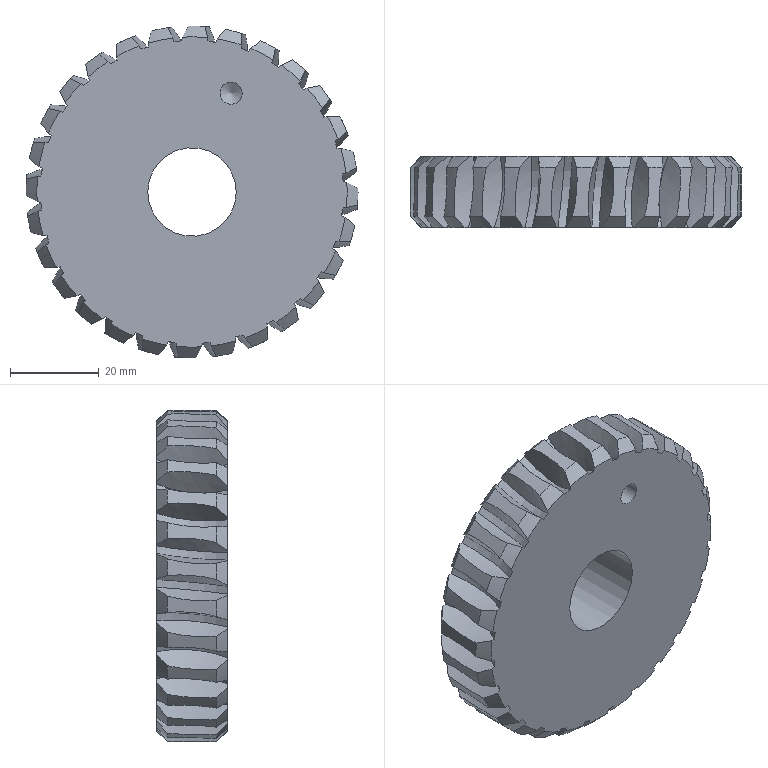Component | NX | WORM_WHEEL | 1 solid | 173 faces | volume 57485 mm3 | spline 84 | cone 57 | cylinder 30 | plane 2 | commonest cylinder face diameters 75 x28 5 x1 20 x1